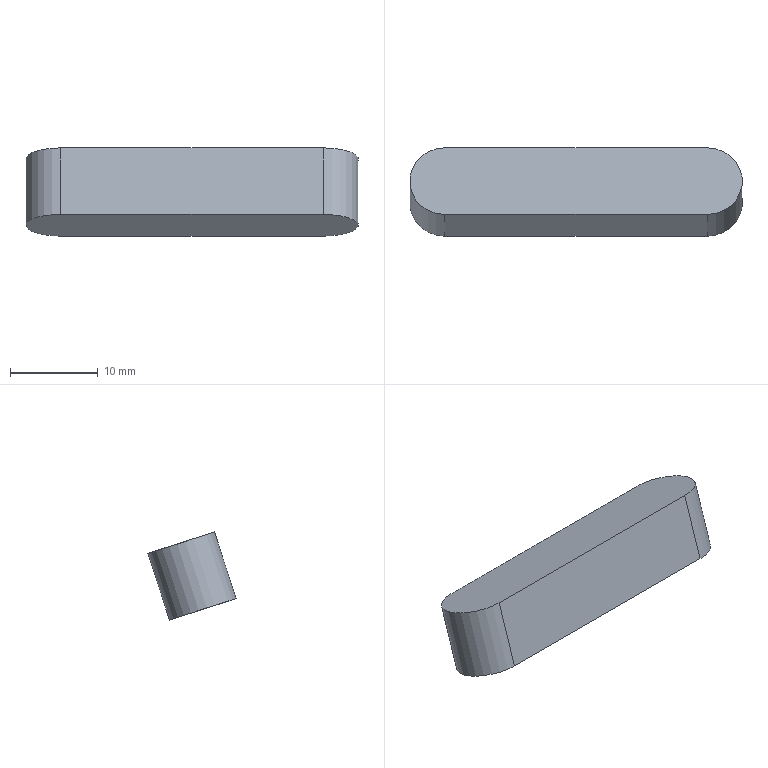Component | NX | PINGJIAN8_2 | 1 solid | 6 faces | box 38 x 10.08 x 10.08 mm | volume 2322 mm3 | plane 4 | cylinder 2 | commonest cylinder face diameters 8 x2
STEP:
#1=CARTESIAN_POINT('',(0.,0.,0.));
#2=DIRECTION('',(0.,0.,1.));
#3=DIRECTION('',(1.,0.,0.));
#4=AXIS2_PLACEMENT_3D('',#1,#2,#3);
#5=CARTESIAN_POINT('',(-51.25,95.939,-74.97));
#6=VERTEX_POINT('',#5);
#7=CARTESIAN_POINT('',(-51.25,88.331,-72.498));
#8=VERTEX_POINT('',#7);
#9=CARTESIAN_POINT('',(-51.25,92.135,-73.734));
#10=DIRECTION('',(0.,0.309,0.9511));
#11=DIRECTION('',(1.,0.,0.));
#12=AXIS2_PLACEMENT_3D('',#9,#10,#11);
#13=CIRCLE('',#12,4.);
#14=CARTESIAN_POINT('',(-51.25,94.607,-66.126));
#15=DIRECTION('',(0.,-0.309,-0.9511));
#16=DIRECTION('',(-1.,0.,0.));
#17=AXIS2_PLACEMENT_3D('',#14,#15,#16);
#18=CYLINDRICAL_SURFACE('',#17,4.);
#19=CARTESIAN_POINT('',(3.142,8.));
#20=DIRECTION('',(-1.,0.));
#21=VECTOR('',#20,1.);
#22=LINE('',#19,#21);
#23=(GEOMETRIC_REPRESENTATION_CONTEXT(2)PARAMETRIC_REPRESENTATION_CONTEXT()REPRESENTATION_CONTEXT('',''));
#24=DEFINITIONAL_REPRESENTATION('',(#22),#23);
#25=PCURVE('',#18,#24);
#26=CARTESIAN_POINT('',(-51.25,92.135,-73.734));
#27=DIRECTION('',(0.,0.309,0.9511));
#28=DIRECTION('',(1.,0.,0.));
#29=AXIS2_PLACEMENT_3D('',#26,#27,#28);
#30=PLANE('',#29);
#31=CARTESIAN_POINT('',(0.,0.));
#32=DIRECTION('',(1.,0.));
#33=AXIS2_PLACEMENT_2D('',#31,#32);
#34=CIRCLE('',#33,4.);
#35=(GEOMETRIC_REPRESENTATION_CONTEXT(2)PARAMETRIC_REPRESENTATION_CONTEXT()REPRESENTATION_CONTEXT('',''));
#36=DEFINITIONAL_REPRESENTATION('',(#34),#35);
#37=PCURVE('',#30,#36);
#38=SURFACE_CURVE('',#13,(#25,#37),.PCURVE_S1.);
#39=EDGE_CURVE('',#6,#8,#38,.T.);
#40=ORIENTED_EDGE('',*,*,#39,.T.);
#41=CARTESIAN_POINT('',(-51.25,90.803,-64.89));
#42=VERTEX_POINT('',#41);
#43=CARTESIAN_POINT('',(-51.25,90.803,-64.89));
#44=DIRECTION('',(0.,-0.309,-0.9511));
#45=VECTOR('',#44,1.);
#46=LINE('',#43,#45);
#47=CARTESIAN_POINT('',(-1.571,-0.));
#48=DIRECTION('',(0.,1.));
#49=VECTOR('',#48,1.);
#50=LINE('',#47,#49);
#51=(GEOMETRIC_REPRESENTATION_CONTEXT(2)PARAMETRIC_REPRESENTATION_CONTEXT()REPRESENTATION_CONTEXT('',''));
#52=DEFINITIONAL_REPRESENTATION('',(#50),#51);
#53=PCURVE('',#18,#52);
#54=CARTESIAN_POINT('',(-51.25,90.803,-64.89));
#55=DIRECTION('',(0.,0.9511,-0.309));
#56=DIRECTION('',(0.,0.309,0.9511));
#57=AXIS2_PLACEMENT_3D('',#54,#55,#56);
#58=PLANE('',#57);
#59=CARTESIAN_POINT('',(0.,0.));
#60=DIRECTION('',(-1.,0.));
#61=VECTOR('',#60,1.);
#62=LINE('',#59,#61);
#63=(GEOMETRIC_REPRESENTATION_CONTEXT(2)PARAMETRIC_REPRESENTATION_CONTEXT()REPRESENTATION_CONTEXT('',''));
#64=DEFINITIONAL_REPRESENTATION('',(#62),#63);
#65=PCURVE('',#58,#64);
#66=SURFACE_CURVE('',#46,(#53,#65),.PCURVE_S1.);
#67=EDGE_CURVE('',#42,#8,#66,.T.);
#68=ORIENTED_EDGE('',*,*,#67,.F.);
#69=CARTESIAN_POINT('',(-51.25,98.412,-67.362));
#70=VERTEX_POINT('',#69);
#71=CARTESIAN_POINT('',(-51.25,94.607,-66.126));
#72=DIRECTION('',(0.,0.309,0.9511));
#73=DIRECTION('',(1.,0.,0.));
#74=AXIS2_PLACEMENT_3D('',#71,#72,#73);
#75=CIRCLE('',#74,4.);
#76=CARTESIAN_POINT('',(3.142,0.));
#77=DIRECTION('',(-1.,0.));
#78=VECTOR('',#77,1.);
#79=LINE('',#76,#78);
#80=(GEOMETRIC_REPRESENTATION_CONTEXT(2)PARAMETRIC_REPRESENTATION_CONTEXT()REPRESENTATION_CONTEXT('',''));
#81=DEFINITIONAL_REPRESENTATION('',(#79),#80);
#82=PCURVE('',#18,#81);
#83=CARTESIAN_POINT('',(-51.25,94.607,-66.126));
#84=DIRECTION('',(0.,0.309,0.9511));
#85=DIRECTION('',(1.,0.,0.));
#86=AXIS2_PLACEMENT_3D('',#83,#84,#85);
#87=PLANE('',#86);
#88=CARTESIAN_POINT('',(0.,0.));
#89=DIRECTION('',(1.,0.));
#90=AXIS2_PLACEMENT_2D('',#88,#89);
#91=CIRCLE('',#90,4.);
#92=(GEOMETRIC_REPRESENTATION_CONTEXT(2)PARAMETRIC_REPRESENTATION_CONTEXT()REPRESENTATION_CONTEXT('',''));
#93=DEFINITIONAL_REPRESENTATION('',(#91),#92);
#94=PCURVE('',#87,#93);
#95=SURFACE_CURVE('',#75,(#82,#94),.PCURVE_S1.);
#96=EDGE_CURVE('',#70,#42,#95,.T.);
#97=ORIENTED_EDGE('',*,*,#96,.F.);
#98=CARTESIAN_POINT('',(-51.25,98.412,-67.362));
#99=DIRECTION('',(0.,-0.309,-0.9511));
#100=VECTOR('',#99,1.);
#101=LINE('',#98,#100);
#102=CARTESIAN_POINT('',(1.571,-0.));
#103=DIRECTION('',(0.,1.));
#104=VECTOR('',#103,1.);
#105=LINE('',#102,#104);
#106=(GEOMETRIC_REPRESENTATION_CONTEXT(2)PARAMETRIC_REPRESENTATION_CONTEXT()REPRESENTATION_CONTEXT('',''));
#107=DEFINITIONAL_REPRESENTATION('',(#105),#106);
#108=PCURVE('',#18,#107);
#109=CARTESIAN_POINT('',(-21.25,98.412,-67.362));
#110=DIRECTION('',(0.,-0.9511,0.309));
#111=DIRECTION('',(0.,-0.309,-0.9511));
#112=AXIS2_PLACEMENT_3D('',#109,#110,#111);
#113=PLANE('',#112);
#114=CARTESIAN_POINT('',(0.,-30.));
#115=DIRECTION('',(1.,0.));
#116=VECTOR('',#115,1.);
#117=LINE('',#114,#116);
#118=(GEOMETRIC_REPRESENTATION_CONTEXT(2)PARAMETRIC_REPRESENTATION_CONTEXT()REPRESENTATION_CONTEXT('',''));
#119=DEFINITIONAL_REPRESENTATION('',(#117),#118);
#120=PCURVE('',#113,#119);
#121=SURFACE_CURVE('',#101,(#108,#120),.PCURVE_S1.);
#122=EDGE_CURVE('',#70,#6,#121,.T.);
#123=ORIENTED_EDGE('',*,*,#122,.T.);
#124=EDGE_LOOP('',(#40,#68,#97,#123));
#125=FACE_BOUND('',#124,.T.);
#126=ADVANCED_FACE('',(#125),#18,.T.);
#127=CARTESIAN_POINT('',(-21.25,88.331,-72.498));
#128=VERTEX_POINT('',#127);
#129=CARTESIAN_POINT('',(-51.25,88.331,-72.498));
#130=DIRECTION('',(1.,0.,0.));
#131=VECTOR('',#130,1.);
#132=LINE('',#129,#131);
#133=CARTESIAN_POINT('',(-8.,0.));
#134=DIRECTION('',(0.,1.));
#135=VECTOR('',#134,1.);
#136=LINE('',#133,#135);
#137=(GEOMETRIC_REPRESENTATION_CONTEXT(2)PARAMETRIC_REPRESENTATION_CONTEXT()REPRESENTATION_CONTEXT('',''));
#138=DEFINITIONAL_REPRESENTATION('',(#136),#137);
#139=PCURVE('',#58,#138);
#140=CARTESIAN_POINT('',(0.,-4.));
#141=DIRECTION('',(1.,0.));
#142=VECTOR('',#141,1.);
#143=LINE('',#140,#142);
#144=(GEOMETRIC_REPRESENTATION_CONTEXT(2)PARAMETRIC_REPRESENTATION_CONTEXT()REPRESENTATION_CONTEXT('',''));
#145=DEFINITIONAL_REPRESENTATION('',(#143),#144);
#146=PCURVE('',#30,#145);
#147=SURFACE_CURVE('',#132,(#139,#146),.PCURVE_S1.);
#148=EDGE_CURVE('',#8,#128,#147,.T.);
#149=ORIENTED_EDGE('',*,*,#148,.T.);
#150=CARTESIAN_POINT('',(-21.25,90.803,-64.89));
#151=VERTEX_POINT('',#150);
#152=CARTESIAN_POINT('',(-21.25,90.803,-64.89));
#153=DIRECTION('',(0.,-0.309,-0.9511));
#154=VECTOR('',#153,1.);
#155=LINE('',#152,#154);
#156=CARTESIAN_POINT('',(0.,30.));
#157=DIRECTION('',(-1.,0.));
#158=VECTOR('',#157,1.);
#159=LINE('',#156,#158);
#160=(GEOMETRIC_REPRESENTATION_CONTEXT(2)PARAMETRIC_REPRESENTATION_CONTEXT()REPRESENTATION_CONTEXT('',''));
#161=DEFINITIONAL_REPRESENTATION('',(#159),#160);
#162=PCURVE('',#58,#161);
#163=CARTESIAN_POINT('',(-21.25,94.607,-66.126));
#164=DIRECTION('',(0.,-0.309,-0.9511));
#165=DIRECTION('',(-1.,0.,0.));
#166=AXIS2_PLACEMENT_3D('',#163,#164,#165);
#167=CYLINDRICAL_SURFACE('',#166,4.);
#168=CARTESIAN_POINT('',(4.712,-0.));
#169=DIRECTION('',(0.,1.));
#170=VECTOR('',#169,1.);
#171=LINE('',#168,#170);
#172=(GEOMETRIC_REPRESENTATION_CONTEXT(2)PARAMETRIC_REPRESENTATION_CONTEXT()REPRESENTATION_CONTEXT('',''));
#173=DEFINITIONAL_REPRESENTATION('',(#171),#172);
#174=PCURVE('',#167,#173);
#175=SURFACE_CURVE('',#155,(#162,#174),.PCURVE_S1.);
#176=EDGE_CURVE('',#151,#128,#175,.T.);
#177=ORIENTED_EDGE('',*,*,#176,.F.);
#178=CARTESIAN_POINT('',(-51.25,90.803,-64.89));
#179=DIRECTION('',(1.,0.,0.));
#180=VECTOR('',#179,1.);
#181=LINE('',#178,#180);
#182=CARTESIAN_POINT('',(0.,0.));
#183=DIRECTION('',(0.,1.));
#184=VECTOR('',#183,1.);
#185=LINE('',#182,#184);
#186=(GEOMETRIC_REPRESENTATION_CONTEXT(2)PARAMETRIC_REPRESENTATION_CONTEXT()REPRESENTATION_CONTEXT('',''));
#187=DEFINITIONAL_REPRESENTATION('',(#185),#186);
#188=PCURVE('',#58,#187);
#189=CARTESIAN_POINT('',(0.,-4.));
#190=DIRECTION('',(1.,0.));
#191=VECTOR('',#190,1.);
#192=LINE('',#189,#191);
#193=(GEOMETRIC_REPRESENTATION_CONTEXT(2)PARAMETRIC_REPRESENTATION_CONTEXT()REPRESENTATION_CONTEXT('',''));
#194=DEFINITIONAL_REPRESENTATION('',(#192),#193);
#195=PCURVE('',#87,#194);
#196=SURFACE_CURVE('',#181,(#188,#195),.PCURVE_S1.);
#197=EDGE_CURVE('',#42,#151,#196,.T.);
#198=ORIENTED_EDGE('',*,*,#197,.F.);
#199=ORIENTED_EDGE('',*,*,#67,.T.);
#200=EDGE_LOOP('',(#149,#177,#198,#199));
#201=FACE_BOUND('',#200,.T.);
#202=ADVANCED_FACE('',(#201),#58,.F.);
#203=CARTESIAN_POINT('',(-21.25,95.939,-74.97));
#204=VERTEX_POINT('',#203);
#205=CARTESIAN_POINT('',(-21.25,92.135,-73.734));
#206=DIRECTION('',(0.,0.309,0.9511));
#207=DIRECTION('',(1.,0.,0.));
#208=AXIS2_PLACEMENT_3D('',#205,#206,#207);
#209=CIRCLE('',#208,4.);
#210=CARTESIAN_POINT('',(9.425,8.));
#211=DIRECTION('',(-1.,0.));
#212=VECTOR('',#211,1.);
#213=LINE('',#210,#212);
#214=(GEOMETRIC_REPRESENTATION_CONTEXT(2)PARAMETRIC_REPRESENTATION_CONTEXT()REPRESENTATION_CONTEXT('',''));
#215=DEFINITIONAL_REPRESENTATION('',(#213),#214);
#216=PCURVE('',#167,#215);
#217=CARTESIAN_POINT('',(30.,0.));
#218=DIRECTION('',(1.,0.));
#219=AXIS2_PLACEMENT_2D('',#217,#218);
#220=CIRCLE('',#219,4.);
#221=(GEOMETRIC_REPRESENTATION_CONTEXT(2)PARAMETRIC_REPRESENTATION_CONTEXT()REPRESENTATION_CONTEXT('',''));
#222=DEFINITIONAL_REPRESENTATION('',(#220),#221);
#223=PCURVE('',#30,#222);
#224=SURFACE_CURVE('',#209,(#216,#223),.PCURVE_S1.);
#225=EDGE_CURVE('',#128,#204,#224,.T.);
#226=ORIENTED_EDGE('',*,*,#225,.T.);
#227=CARTESIAN_POINT('',(-21.25,98.412,-67.362));
#228=VERTEX_POINT('',#227);
#229=CARTESIAN_POINT('',(-21.25,98.412,-67.362));
#230=DIRECTION('',(0.,-0.309,-0.9511));
#231=VECTOR('',#230,1.);
#232=LINE('',#229,#231);
#233=CARTESIAN_POINT('',(1.571,-0.));
#234=DIRECTION('',(0.,1.));
#235=VECTOR('',#234,1.);
#236=LINE('',#233,#235);
#237=(GEOMETRIC_REPRESENTATION_CONTEXT(2)PARAMETRIC_REPRESENTATION_CONTEXT()REPRESENTATION_CONTEXT('',''));
#238=DEFINITIONAL_REPRESENTATION('',(#236),#237);
#239=PCURVE('',#167,#238);
#240=CARTESIAN_POINT('',(0.,0.));
#241=DIRECTION('',(1.,0.));
#242=VECTOR('',#241,1.);
#243=LINE('',#240,#242);
#244=(GEOMETRIC_REPRESENTATION_CONTEXT(2)PARAMETRIC_REPRESENTATION_CONTEXT()REPRESENTATION_CONTEXT('',''));
#245=DEFINITIONAL_REPRESENTATION('',(#243),#244);
#246=PCURVE('',#113,#245);
#247=SURFACE_CURVE('',#232,(#239,#246),.PCURVE_S1.);
#248=EDGE_CURVE('',#228,#204,#247,.T.);
#249=ORIENTED_EDGE('',*,*,#248,.F.);
#250=CARTESIAN_POINT('',(-21.25,94.607,-66.126));
#251=DIRECTION('',(0.,0.309,0.9511));
#252=DIRECTION('',(1.,0.,0.));
#253=AXIS2_PLACEMENT_3D('',#250,#251,#252);
#254=CIRCLE('',#253,4.);
#255=CARTESIAN_POINT('',(9.425,0.));
#256=DIRECTION('',(-1.,0.));
#257=VECTOR('',#256,1.);
#258=LINE('',#255,#257);
#259=(GEOMETRIC_REPRESENTATION_CONTEXT(2)PARAMETRIC_REPRESENTATION_CONTEXT()REPRESENTATION_CONTEXT('',''));
#260=DEFINITIONAL_REPRESENTATION('',(#258),#259);
#261=PCURVE('',#167,#260);
#262=CARTESIAN_POINT('',(30.,0.));
#263=DIRECTION('',(1.,0.));
#264=AXIS2_PLACEMENT_2D('',#262,#263);
#265=CIRCLE('',#264,4.);
#266=(GEOMETRIC_REPRESENTATION_CONTEXT(2)PARAMETRIC_REPRESENTATION_CONTEXT()REPRESENTATION_CONTEXT('',''));
#267=DEFINITIONAL_REPRESENTATION('',(#265),#266);
#268=PCURVE('',#87,#267);
#269=SURFACE_CURVE('',#254,(#261,#268),.PCURVE_S1.);
#270=EDGE_CURVE('',#151,#228,#269,.T.);
#271=ORIENTED_EDGE('',*,*,#270,.F.);
#272=ORIENTED_EDGE('',*,*,#176,.T.);
#273=EDGE_LOOP('',(#226,#249,#271,#272));
#274=FACE_BOUND('',#273,.T.);
#275=ADVANCED_FACE('',(#274),#167,.T.);
#276=CARTESIAN_POINT('',(-21.25,95.939,-74.97));
#277=DIRECTION('',(-1.,0.,0.));
#278=VECTOR('',#277,1.);
#279=LINE('',#276,#278);
#280=CARTESIAN_POINT('',(8.,0.));
#281=DIRECTION('',(0.,-1.));
#282=VECTOR('',#281,1.);
#283=LINE('',#280,#282);
#284=(GEOMETRIC_REPRESENTATION_CONTEXT(2)PARAMETRIC_REPRESENTATION_CONTEXT()REPRESENTATION_CONTEXT('',''));
#285=DEFINITIONAL_REPRESENTATION('',(#283),#284);
#286=PCURVE('',#113,#285);
#287=CARTESIAN_POINT('',(30.,4.));
#288=DIRECTION('',(-1.,0.));
#289=VECTOR('',#288,1.);
#290=LINE('',#287,#289);
#291=(GEOMETRIC_REPRESENTATION_CONTEXT(2)PARAMETRIC_REPRESENTATION_CONTEXT()REPRESENTATION_CONTEXT('',''));
#292=DEFINITIONAL_REPRESENTATION('',(#290),#291);
#293=PCURVE('',#30,#292);
#294=SURFACE_CURVE('',#279,(#286,#293),.PCURVE_S1.);
#295=EDGE_CURVE('',#204,#6,#294,.T.);
#296=ORIENTED_EDGE('',*,*,#295,.T.);
#297=ORIENTED_EDGE('',*,*,#122,.F.);
#298=CARTESIAN_POINT('',(-21.25,98.412,-67.362));
#299=DIRECTION('',(-1.,0.,0.));
#300=VECTOR('',#299,1.);
#301=LINE('',#298,#300);
#302=CARTESIAN_POINT('',(0.,0.));
#303=DIRECTION('',(0.,-1.));
#304=VECTOR('',#303,1.);
#305=LINE('',#302,#304);
#306=(GEOMETRIC_REPRESENTATION_CONTEXT(2)PARAMETRIC_REPRESENTATION_CONTEXT()REPRESENTATION_CONTEXT('',''));
#307=DEFINITIONAL_REPRESENTATION('',(#305),#306);
#308=PCURVE('',#113,#307);
#309=CARTESIAN_POINT('',(30.,4.));
#310=DIRECTION('',(-1.,0.));
#311=VECTOR('',#310,1.);
#312=LINE('',#309,#311);
#313=(GEOMETRIC_REPRESENTATION_CONTEXT(2)PARAMETRIC_REPRESENTATION_CONTEXT()REPRESENTATION_CONTEXT('',''));
#314=DEFINITIONAL_REPRESENTATION('',(#312),#313);
#315=PCURVE('',#87,#314);
#316=SURFACE_CURVE('',#301,(#308,#315),.PCURVE_S1.);
#317=EDGE_CURVE('',#228,#70,#316,.T.);
#318=ORIENTED_EDGE('',*,*,#317,.F.);
#319=ORIENTED_EDGE('',*,*,#248,.T.);
#320=EDGE_LOOP('',(#296,#297,#318,#319));
#321=FACE_BOUND('',#320,.T.);
#322=ADVANCED_FACE('',(#321),#113,.F.);
#323=ORIENTED_EDGE('',*,*,#96,.T.);
#324=ORIENTED_EDGE('',*,*,#197,.T.);
#325=ORIENTED_EDGE('',*,*,#270,.T.);
#326=ORIENTED_EDGE('',*,*,#317,.T.);
#327=EDGE_LOOP('',(#323,#324,#325,#326));
#328=FACE_BOUND('',#327,.T.);
#329=ADVANCED_FACE('',(#328),#87,.T.);
#330=ORIENTED_EDGE('',*,*,#39,.F.);
#331=ORIENTED_EDGE('',*,*,#295,.F.);
#332=ORIENTED_EDGE('',*,*,#225,.F.);
#333=ORIENTED_EDGE('',*,*,#148,.F.);
#334=EDGE_LOOP('',(#330,#331,#332,#333));
#335=FACE_BOUND('',#334,.T.);
#336=ADVANCED_FACE('',(#335),#30,.F.);
#337=CLOSED_SHELL('',(#126,#202,#275,#322,#329,#336));
#338=MANIFOLD_SOLID_BREP('',#337);
#339=(LENGTH_UNIT()NAMED_UNIT(*)SI_UNIT(.MILLI.,.METRE.));
#340=UNCERTAINTY_MEASURE_WITH_UNIT(LENGTH_MEASURE(0.0000001),#339,'','');
#341=(NAMED_UNIT(*)PLANE_ANGLE_UNIT()SI_UNIT($,.RADIAN.));
#342=(NAMED_UNIT(*)SI_UNIT($,.STERADIAN.)SOLID_ANGLE_UNIT());
#343=(GEOMETRIC_REPRESENTATION_CONTEXT(3)GLOBAL_UNCERTAINTY_ASSIGNED_CONTEXT((#340))GLOBAL_UNIT_ASSIGNED_CONTEXT((#339,#341,#342))REPRESENTATION_CONTEXT('',''));
#344=ADVANCED_BREP_SHAPE_REPRESENTATION('',(#4,#338),#343);